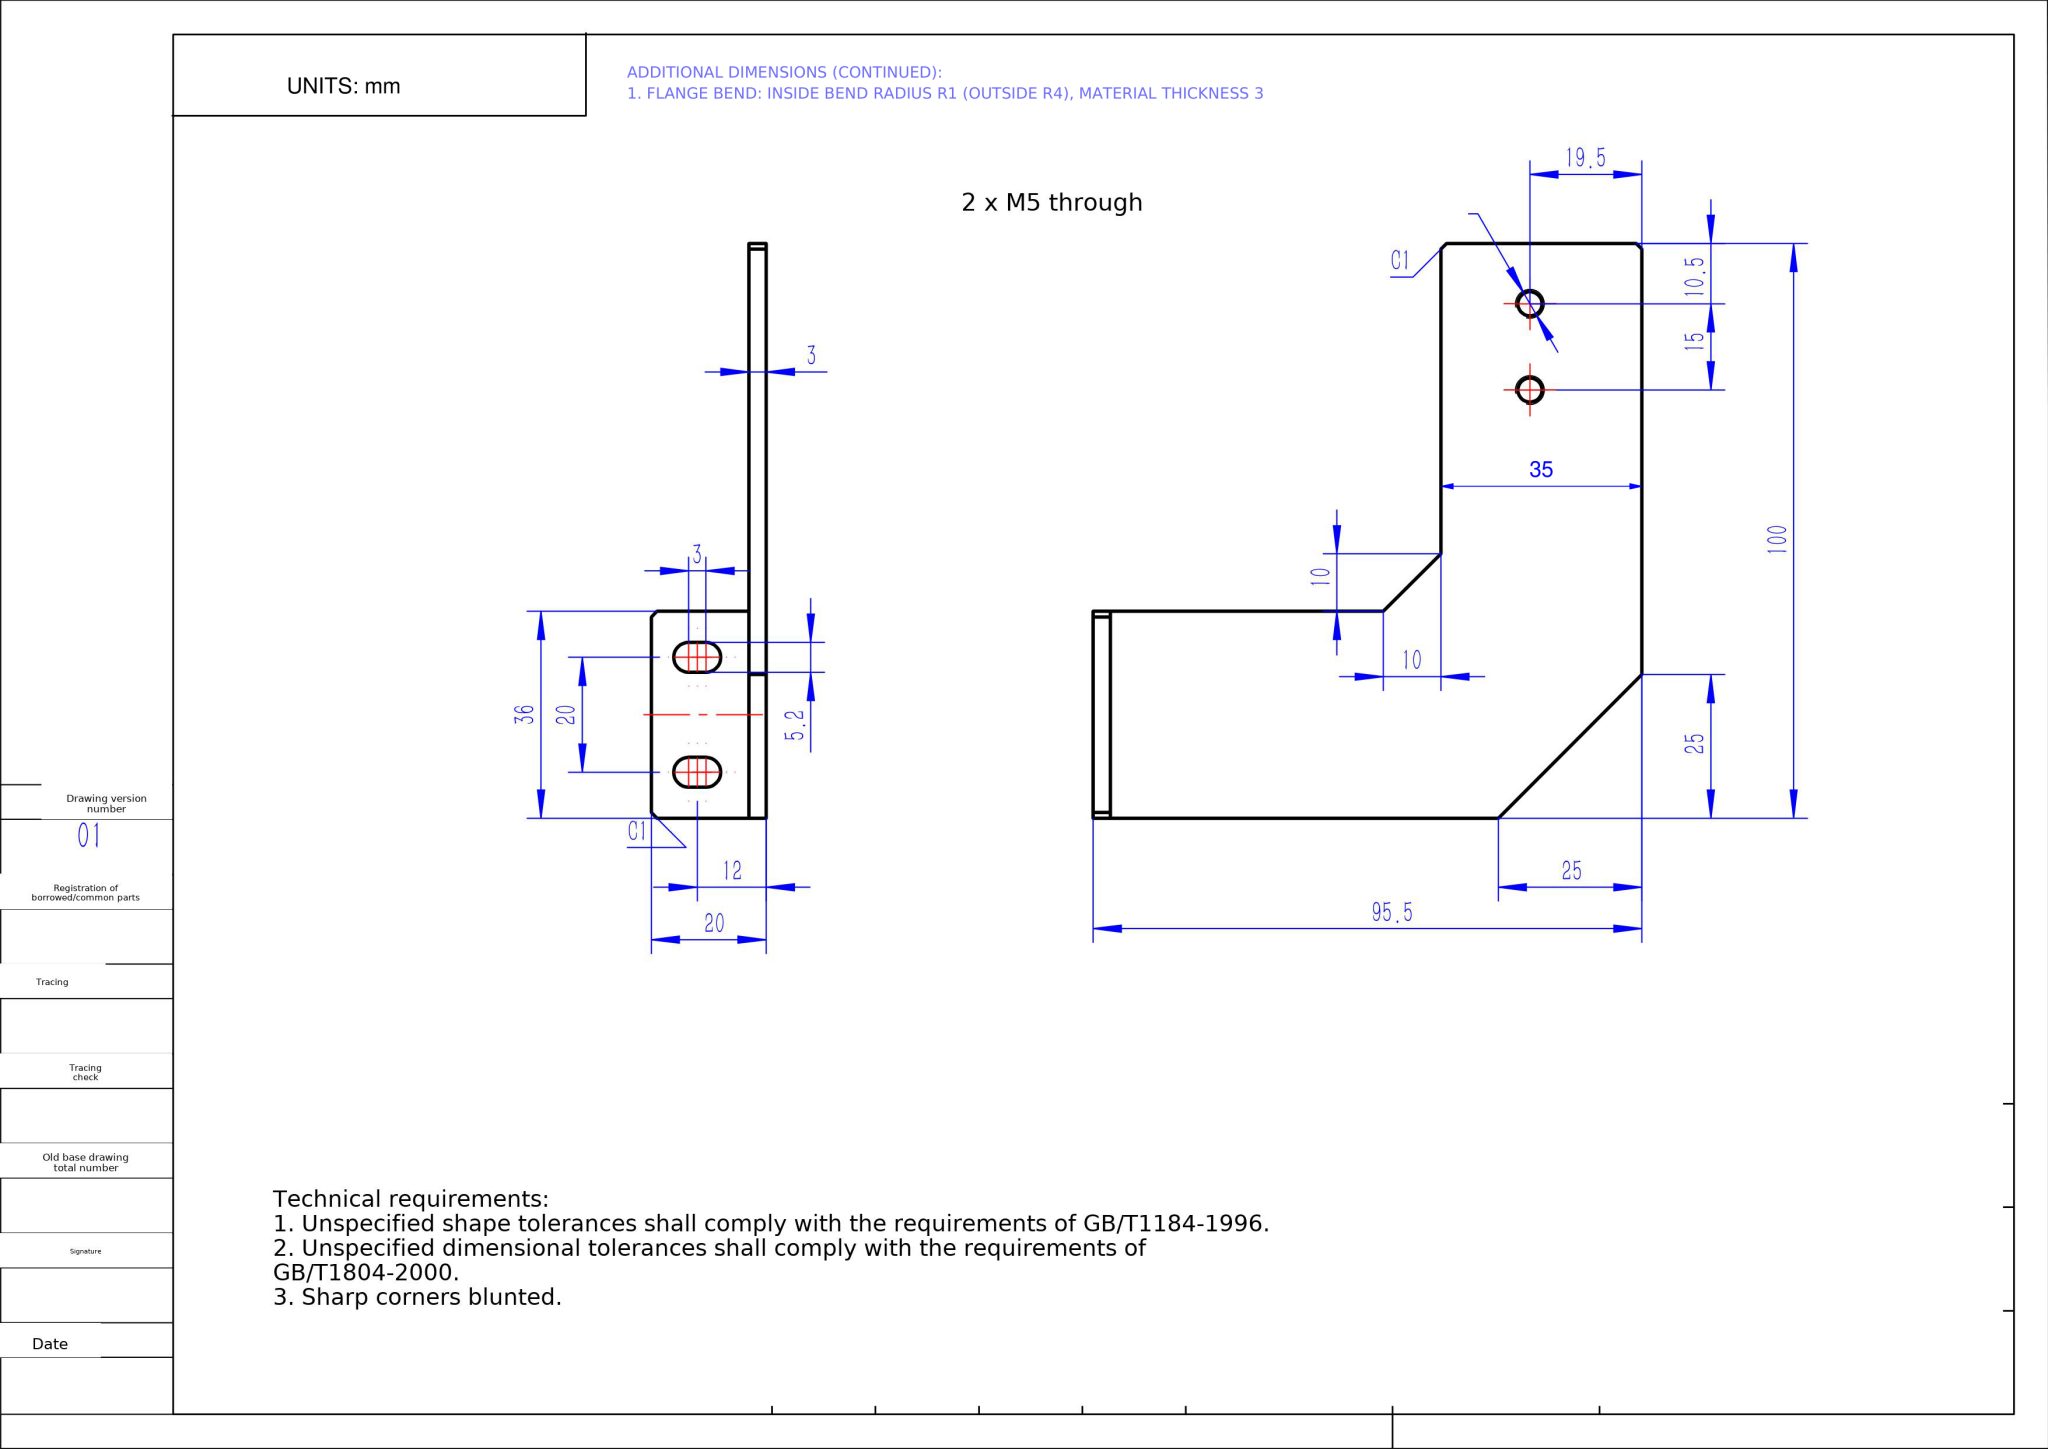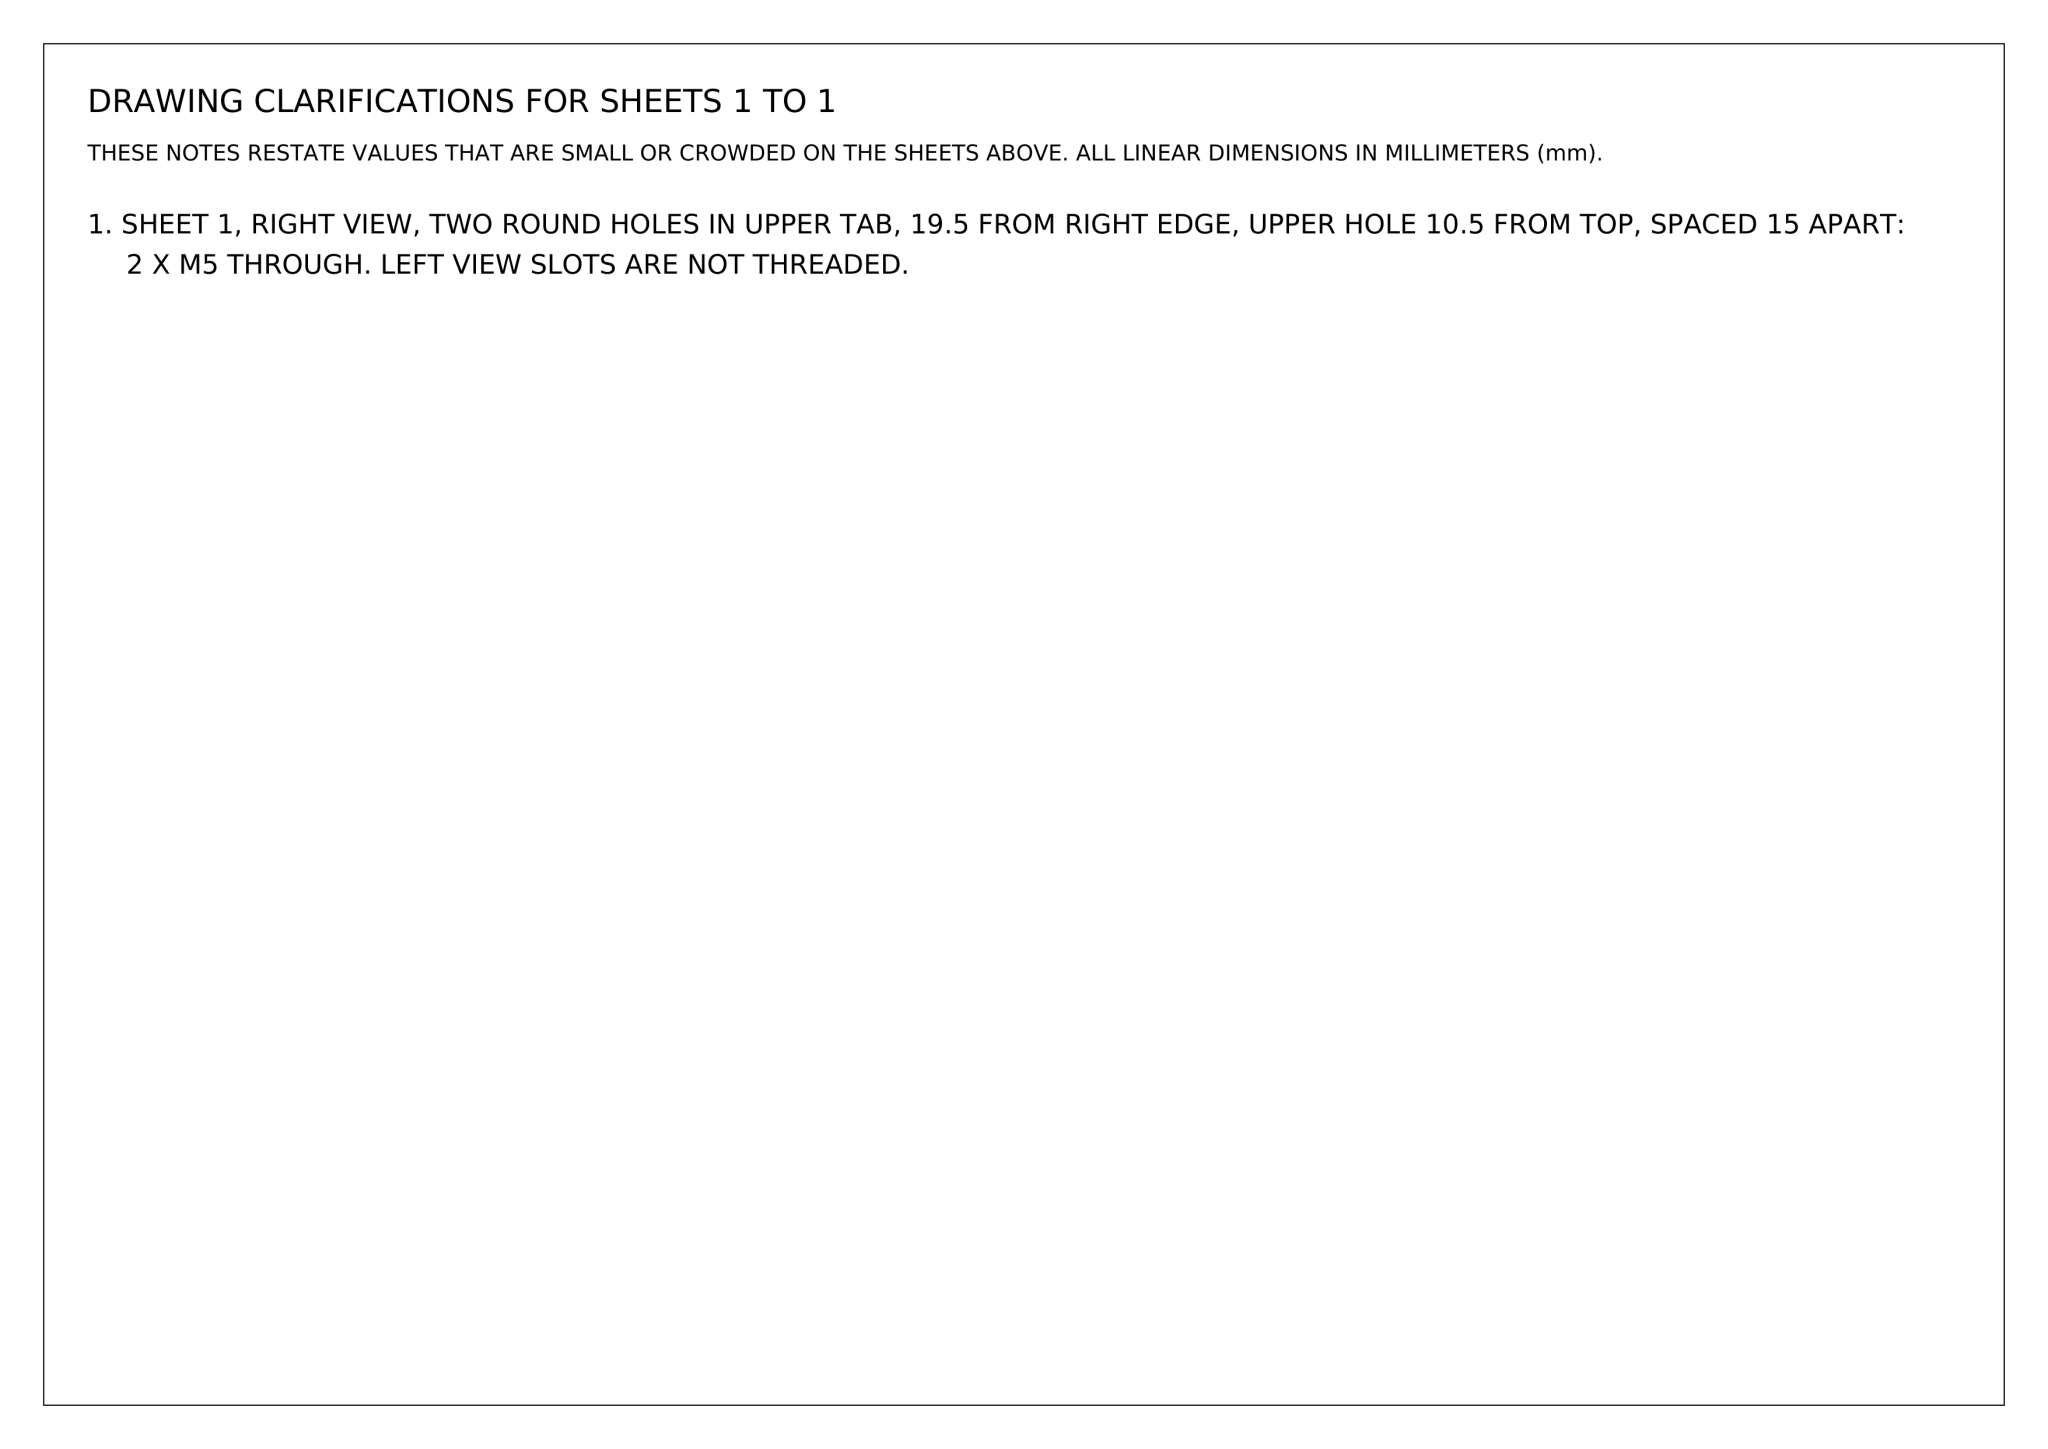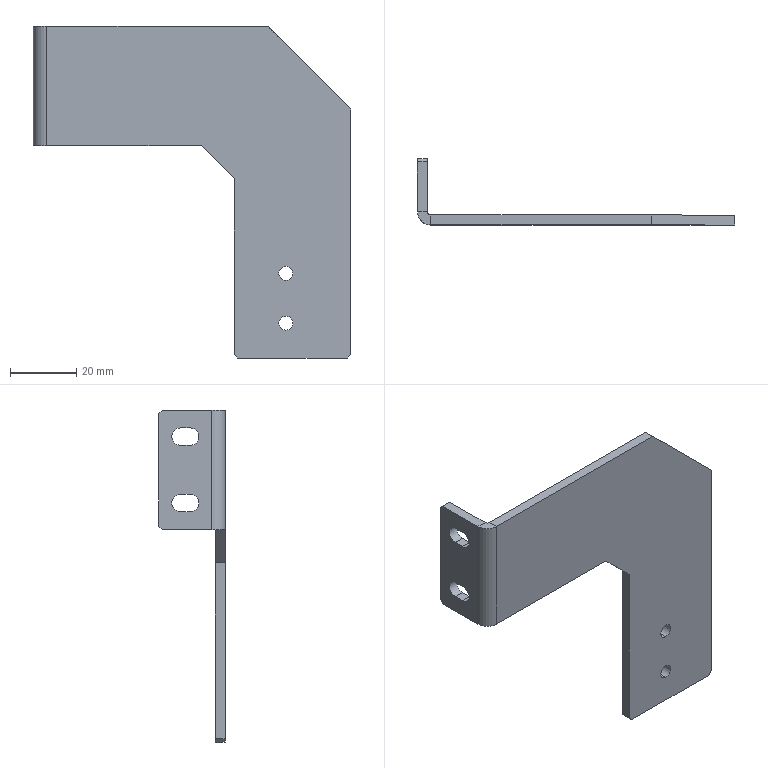Part | NX | mm | 1 solid | 32 faces | box 95.5 x 20 x 100 mm | volume 17656 mm3 | plane 22 | cylinder 10 | commonest cylinder face diameters 4.2 x4 5.2 x4 8 x1 2 x1